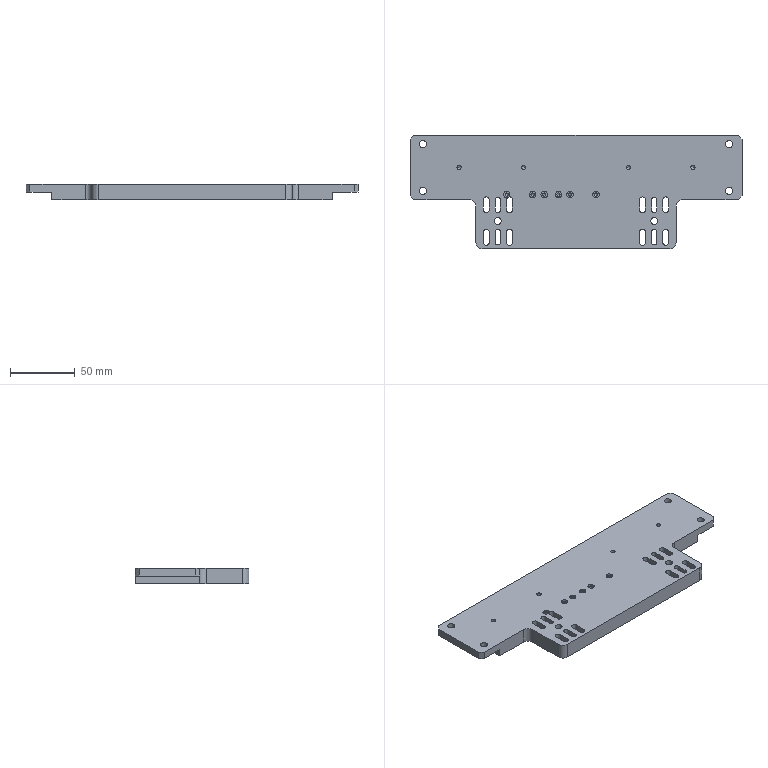Component | SolidWorks | 02-1111-4 | 1 solid | 161 faces | box 257 x 88 x 12 mm | volume 202297 mm3 | cylinder 83 | plane 48 | cone 30 | commonest cylinder face diameters 5 x19 4.5 x16 2.5 x12 5.5 x12 3.3 x8 4 x8 6 x4 10 x4
build123d program:
from build123d import *

# Parameters (mm, degrees)
SKETCH5_W                      = 50
SKETCH5_H                      = 257
BOSS_EXTRUDE1_DEPTH            = 12
SKETCH6_W                      = 50
SKETCH6_H                      = 20
CUT_EXTRUDE4_DEPTH             = 6
SKETCH8_W                      = 155
SKETCH8_H                      = 12
BOSS_EXTRUDE2_DEPTH            = 38
FILLET2_R                      = 5
SKETCH9_R                      = 2.75
CUT_EXTRUDE6_DEPTH             = 144.615
CUT_EXTRUDE7_DEPTH             = 144.615
M5_CLEARANCE_HOLE1_AT_2_COUNT  = 2
M5_CLEARANCE_HOLE1_AT_2_PITCH  = 36
CHAMFER1_SIZE                  = 3
M3_TAPPED_HOLE1_D              = 2.5
M3_TAPPED_HOLE1_DEPTH          = 7.5
M3_TAPPED_HOLE1_TIP            = 0.7511
M3_TAPPED_HOLE2_D              = 2.5
M3_TAPPED_HOLE2_DEPTH          = 7.5
M3_TAPPED_HOLE2_TIP            = 0.7511
SKETCH17_R                     = 2.5
CUT_EXTRUDE8_DEPTH             = 1.3
LPATTERN1_COUNT                = 2
LPATTERN1_PITCH                = 50
M6_TAPPED_HOLE1_D              = 5
M6_TAPPED_HOLE1_DEPTH          = 15
M6_TAPPED_HOLE1_TIP            = 1.502
SIZE_MM_DOWEL_PIN_HOLE_1_D     = 6
SIZE_MM_DOWEL_PIN_HOLE_1_DEPTH = 10
SIZE_MM_DOWEL_PIN_HOLE_1_TIP   = 1.803
M6_TAPPED_HOLE2_D              = 5
M6_TAPPED_HOLE2_DEPTH          = 15
M6_TAPPED_HOLE2_TIP            = 1.502
SIZE_MM_DOWEL_PIN_HOLE_2_D     = 6
SIZE_MM_DOWEL_PIN_HOLE_2_DEPTH = 10
SIZE_MM_DOWEL_PIN_HOLE_2_TIP   = 1.803


with BuildPart() as part:
    # Sketch5 → Boss-Extrude1 (new body)
    with BuildSketch(Plane(origin=(0, 0, 0), x_dir=(1, 0, 0), z_dir=(0, 1, 0))):
        Rectangle(SKETCH5_W, SKETCH5_H)
    extrude(amount=BOSS_EXTRUDE1_DEPTH)

    # Sketch6 → Cut-Extrude4 (cut)
    with BuildSketch(Plane(origin=(0, 12, 0), x_dir=(1, 0, 0), z_dir=(0, 1, 0))):
        with Locations((0, -118.5)):
            Rectangle(SKETCH6_W, SKETCH6_H)
        with Locations((0, 118.5)):
            Rectangle(SKETCH6_W, SKETCH6_H)
    extrude(amount=-CUT_EXTRUDE4_DEPTH, mode=Mode.SUBTRACT)

    # Sketch8 → Boss-Extrude2 (add)
    with BuildSketch(Plane.ZY.offset(25)):
        with Locations((0, 6)):
            Rectangle(SKETCH8_W, SKETCH8_H)
    extrude(amount=BOSS_EXTRUDE2_DEPTH)

    # Fillet2
    fillet2_edges = [part.edges().sort_by_distance(p)[0] for p in [
        (-25, 6, -77.5),
        (-25, 6, 77.5),
        (-63, 6, -77.5),
        (-63, 6, 77.5),
    ]]
    fillet(fillet2_edges, radius=FILLET2_R)

    # Sketch9 → Cut-Extrude6 (cut, through all)
    with BuildSketch(Plane.XZ):
        with Locations(Location((-41.5, 60.5, 0), (0, 0, 270))):
            Circle(SKETCH9_R)
    cut_extrude6 = extrude(amount=-CUT_EXTRUDE6_DEPTH, mode=Mode.SUBTRACT)

    # Sketch10 → Cut-Extrude7 (cut, through all)
    with BuildSketch(Plane.XZ):
        with BuildLine():
            Line((-25, 67.25), (-33, 67.25))
            ThreePointArc((-33, 67.25), (-35.25, 69.5), (-33, 71.75))
            Line((-33, 71.75), (-25, 71.75))
            ThreePointArc((-25, 71.75), (-22.75, 69.5), (-25, 67.25))
        make_face()
        with BuildLine():
            Line((-25, 49.25), (-33, 49.25))
            ThreePointArc((-33, 49.25), (-35.25, 51.5), (-33, 53.75))
            Line((-33, 53.75), (-25, 53.75))
            ThreePointArc((-25, 53.75), (-22.75, 51.5), (-25, 49.25))
        make_face()
        with BuildLine():
            Line((-58, 71.75), (-50, 71.75))
            ThreePointArc((-50, 71.75), (-47.75, 69.5), (-50, 67.25))
            Line((-50, 67.25), (-58, 67.25))
            ThreePointArc((-58, 67.25), (-60.25, 69.5), (-58, 71.75))
        make_face()
        with BuildLine():
            Line((-58, 53.75), (-50, 53.75))
            ThreePointArc((-50, 53.75), (-47.75, 51.5), (-50, 49.25))
            Line((-50, 49.25), (-58, 49.25))
            ThreePointArc((-58, 49.25), (-60.25, 51.5), (-58, 53.75))
        make_face()
        with BuildLine():
            Line((-33, 62.5), (-25, 62.5))
            ThreePointArc((-25, 62.5), (-23, 60.5), (-25, 58.5))
            Line((-25, 58.5), (-33, 58.5))
            ThreePointArc((-33, 58.5), (-35, 60.5), (-33, 62.5))
        make_face()
        with BuildLine():
            Line((-58, 62.5), (-50, 62.5))
            ThreePointArc((-50, 62.5), (-48, 60.5), (-50, 58.5))
            Line((-50, 58.5), (-58, 58.5))
            ThreePointArc((-58, 58.5), (-60, 60.5), (-58, 62.5))
        make_face()
    cut_extrude7 = extrude(amount=-CUT_EXTRUDE7_DEPTH, mode=Mode.SUBTRACT)

    # Mirror1: Cut-Extrude6, Cut-Extrude7 across plane
    add(cut_extrude6.mirror(Plane.XY), mode=Mode.SUBTRACT)
    add(cut_extrude7.mirror(Plane.XY), mode=Mode.SUBTRACT)

    # Sketch12 → M5 Clearance Hole1 (revolve, cut)
    with BuildSketch(Plane(origin=(18, 6, -118.5), x_dir=(0, 0, 1), z_dir=(1, 0, 0))):
        Polygon((0, 0), (0, 9.152), (2.75, 7.5), (2.75, 0), align=None)
    m5_clearance_hole1 = revolve(axis=Axis((18, 12.35, -118.5), (0, -1, 0)), mode=Mode.SUBTRACT)

    # M5 Clearance Hole1 at 2: M5 Clearance Hole1 ×2
    with Locations(*[(-i * M5_CLEARANCE_HOLE1_AT_2_PITCH, 0, 0) for i in range(1, M5_CLEARANCE_HOLE1_AT_2_COUNT)]):
        add(m5_clearance_hole1, mode=Mode.SUBTRACT)

    # Mirror2: M5 Clearance Hole1 across plane
    add(m5_clearance_hole1.mirror(Plane.XY), mode=Mode.SUBTRACT)

    # Mirror2 copy 1 sketch → Mirror2 copy 1 (revolve, cut)
    with BuildSketch(Plane(origin=(-18, 6, 118.5), x_dir=(0, 0, -1), z_dir=(1, 0, 0))):
        Polygon((0, 0), (0, -9.152), (2.75, -7.5), (2.75, 0), align=None)
    revolve(axis=Axis((-18, 12.35, 118.5), (0, 1, 0)), mode=Mode.SUBTRACT)

    # Chamfer1
    chamfer1_edges = [part.edges().sort_by_distance(p)[0] for p in [
        (25, 3, 128.5),
        (-25, 3, 128.5),
        (-25, 3, -128.5),
        (25, 3, -128.5),
    ]]
    chamfer(chamfer1_edges, length=CHAMFER1_SIZE)

    # M3 Tapped Hole1
    with Locations(Plane(origin=(0, 0, 0), x_dir=(-1, 0, 0), z_dir=(0, -1, 0))):
        with Locations((21, -24.6), (21, -4.6), (21, 15.4)):
            Hole(M3_TAPPED_HOLE1_D / 2, depth=M3_TAPPED_HOLE1_DEPTH)
            with Locations((0, 0, -(M3_TAPPED_HOLE1_DEPTH + M3_TAPPED_HOLE1_TIP / 2))):  # 118° drill point
                Cone(0, M3_TAPPED_HOLE1_D / 2, M3_TAPPED_HOLE1_TIP, mode=Mode.SUBTRACT)

    # M3 Tapped Hole2
    with Locations(Plane(origin=(0, 0, 0), x_dir=(-1, 0, 0), z_dir=(0, -1, 0))):
        with Locations((21, -13.6), (21, -33.6), (21, -53.6)):
            Hole(M3_TAPPED_HOLE2_D / 2, depth=M3_TAPPED_HOLE2_DEPTH)
            with Locations((0, 0, -(M3_TAPPED_HOLE2_DEPTH + M3_TAPPED_HOLE2_TIP / 2))):  # 118° drill point
                Cone(0, M3_TAPPED_HOLE2_D / 2, M3_TAPPED_HOLE2_TIP, mode=Mode.SUBTRACT)

    # Sketch17 → Cut-Extrude8 (cut)
    with BuildSketch(Plane.XZ):
        with Locations(Location((-21, 24.6, 0), (0, 0, 270))):
            Circle(SKETCH17_R)
        with Locations(Location((-21, 4.6, 0), (0, 0, 270))):
            Circle(SKETCH17_R)
        with Locations(Location((-21, -15.4, 0), (0, 0, 270))):
            Circle(SKETCH17_R)
        with Locations(Location((-21, 33.6, 0), (0, 0, 270))):
            Circle(SKETCH17_R)
        with Locations(Location((-21, 13.6, 0), (0, 0, 270))):
            Circle(SKETCH17_R)
        with Locations((-21, 53.6)):
            Circle(SKETCH17_R)
    extrude(amount=-CUT_EXTRUDE8_DEPTH, mode=Mode.SUBTRACT)

    # Sketch21 → M4 Tapped Hole2 (revolve, cut)
    with BuildSketch(Plane(origin=(0, 0, -90.5), x_dir=(0, 0, -1), z_dir=(1, 0, 0))):
        Polygon((0, 0), (0, 11.091), (1.65, 10.1), (1.65, 0), align=None)
    m4_tapped_hole2 = revolve(axis=Axis((0, -6.35, -90.5), (0, 1, 0)), mode=Mode.SUBTRACT)

    # LPattern1: M4 Tapped Hole2 ×2
    with Locations(*[(0, 0, i * LPATTERN1_PITCH) for i in range(1, LPATTERN1_COUNT)]):
        add(m4_tapped_hole2, mode=Mode.SUBTRACT)

    # Mirror3: M4 Tapped Hole2 across plane
    add(m4_tapped_hole2.mirror(Plane.XY), mode=Mode.SUBTRACT)

    # Mirror3 copy 1 sketch → Mirror3 copy 1 (revolve, cut)
    with BuildSketch(Plane(origin=(0, 0, 40.5), x_dir=(0, 0, 1), z_dir=(1, 0, 0))):
        Polygon((0, 0), (0, -11.091), (1.65, -10.1), (1.65, 0), align=None)
    revolve(axis=Axis((0, -6.35, 40.5), (0, -1, 0)), mode=Mode.SUBTRACT)

    # M6 Tapped Hole1
    with Locations(Plane(origin=(25, 0, 0), x_dir=(0, 0, -1), z_dir=(1, 0, 0))):
        with Locations((-72, 6), (0, 6), (72, 6)):
            Hole(M6_TAPPED_HOLE1_D / 2, depth=M6_TAPPED_HOLE1_DEPTH)
            with Locations((0, 0, -(M6_TAPPED_HOLE1_DEPTH + M6_TAPPED_HOLE1_TIP / 2))):  # 118° drill point
                Cone(0, M6_TAPPED_HOLE1_D / 2, M6_TAPPED_HOLE1_TIP, mode=Mode.SUBTRACT)

    # Size mm Dowel Pin Hole 1
    with Locations(Plane(origin=(25, 0, 0), x_dir=(0, 0, -1), z_dir=(1, 0, 0))):
        with Locations((-57, 6), (57, 6)):
            Hole(SIZE_MM_DOWEL_PIN_HOLE_1_D / 2, depth=SIZE_MM_DOWEL_PIN_HOLE_1_DEPTH)
            with Locations((0, 0, -(SIZE_MM_DOWEL_PIN_HOLE_1_DEPTH + SIZE_MM_DOWEL_PIN_HOLE_1_TIP / 2))):  # 118° drill point
                Cone(0, SIZE_MM_DOWEL_PIN_HOLE_1_D / 2, SIZE_MM_DOWEL_PIN_HOLE_1_TIP, mode=Mode.SUBTRACT)

    # M6 Tapped Hole2
    with Locations(Plane(origin=(25, 0, 0), x_dir=(0, 0, -1), z_dir=(1, 0, 0))):
        with Locations((-72, 6), (0, 6), (72, 6)):
            Hole(M6_TAPPED_HOLE2_D / 2, depth=M6_TAPPED_HOLE2_DEPTH)
            with Locations((0, 0, -(M6_TAPPED_HOLE2_DEPTH + M6_TAPPED_HOLE2_TIP / 2))):  # 118° drill point
                Cone(0, M6_TAPPED_HOLE2_D / 2, M6_TAPPED_HOLE2_TIP, mode=Mode.SUBTRACT)

    # Size mm Dowel Pin Hole 2
    with Locations(Plane(origin=(25, 0, 0), x_dir=(0, 0, -1), z_dir=(1, 0, 0))):
        with Locations((-57, 6), (57, 6)):
            Hole(SIZE_MM_DOWEL_PIN_HOLE_2_D / 2, depth=SIZE_MM_DOWEL_PIN_HOLE_2_DEPTH)
            with Locations((0, 0, -(SIZE_MM_DOWEL_PIN_HOLE_2_DEPTH + SIZE_MM_DOWEL_PIN_HOLE_2_TIP / 2))):  # 118° drill point
                Cone(0, SIZE_MM_DOWEL_PIN_HOLE_2_D / 2, SIZE_MM_DOWEL_PIN_HOLE_2_TIP, mode=Mode.SUBTRACT)


solid = part.part

# Placed as in the assembly
solid = solid.moved(Location((3.428, 516.224, 1516.056), (-90, -90, 0)))